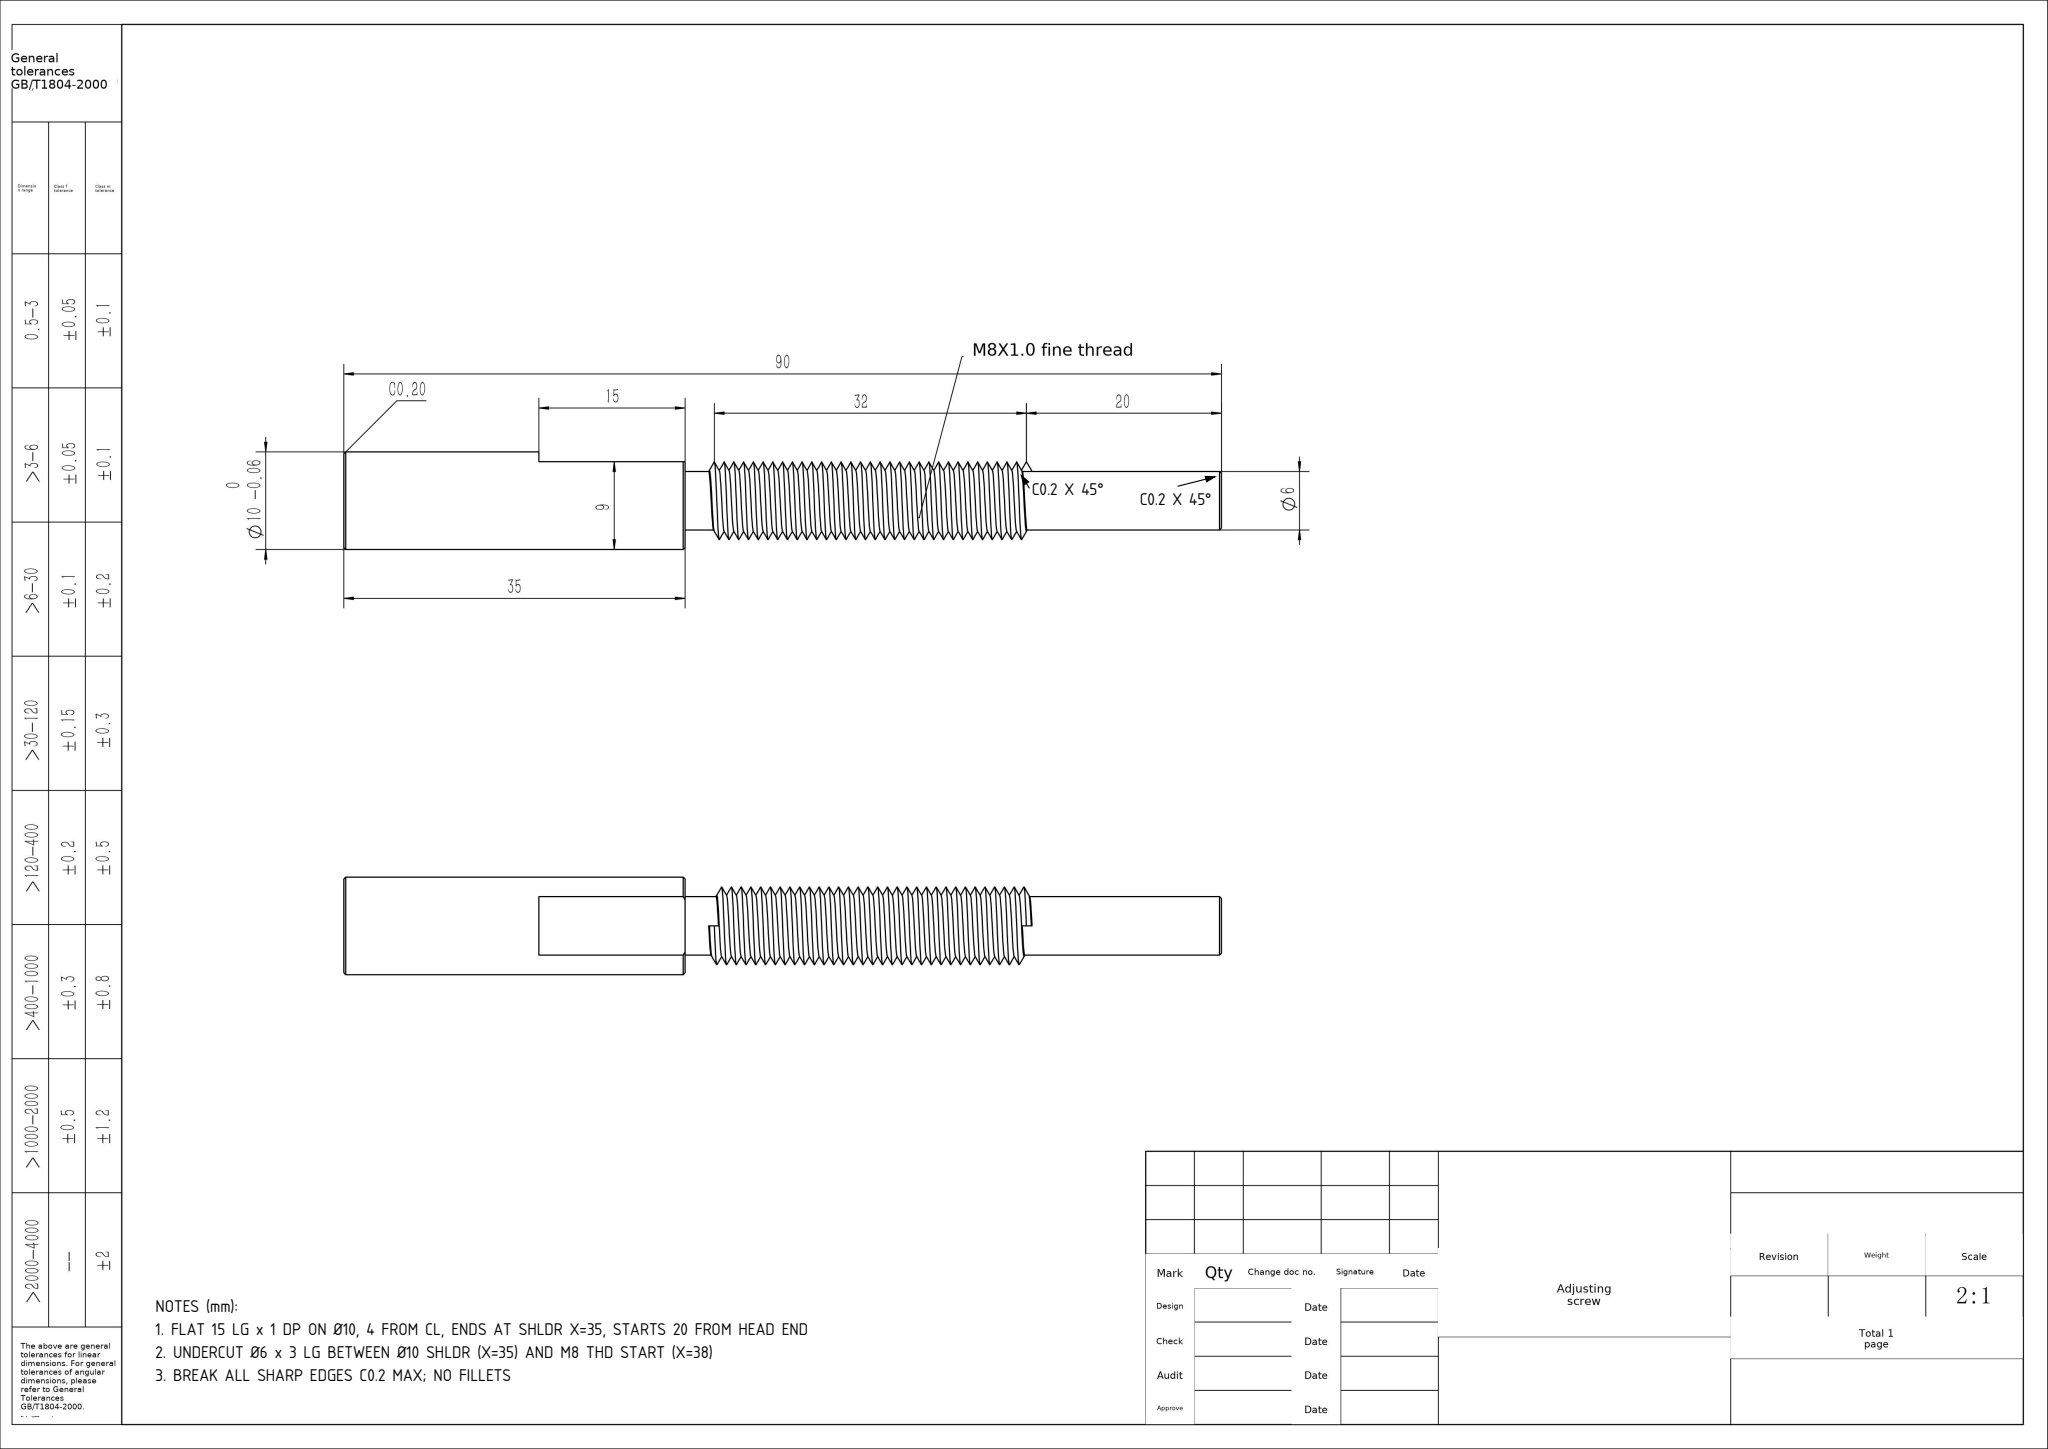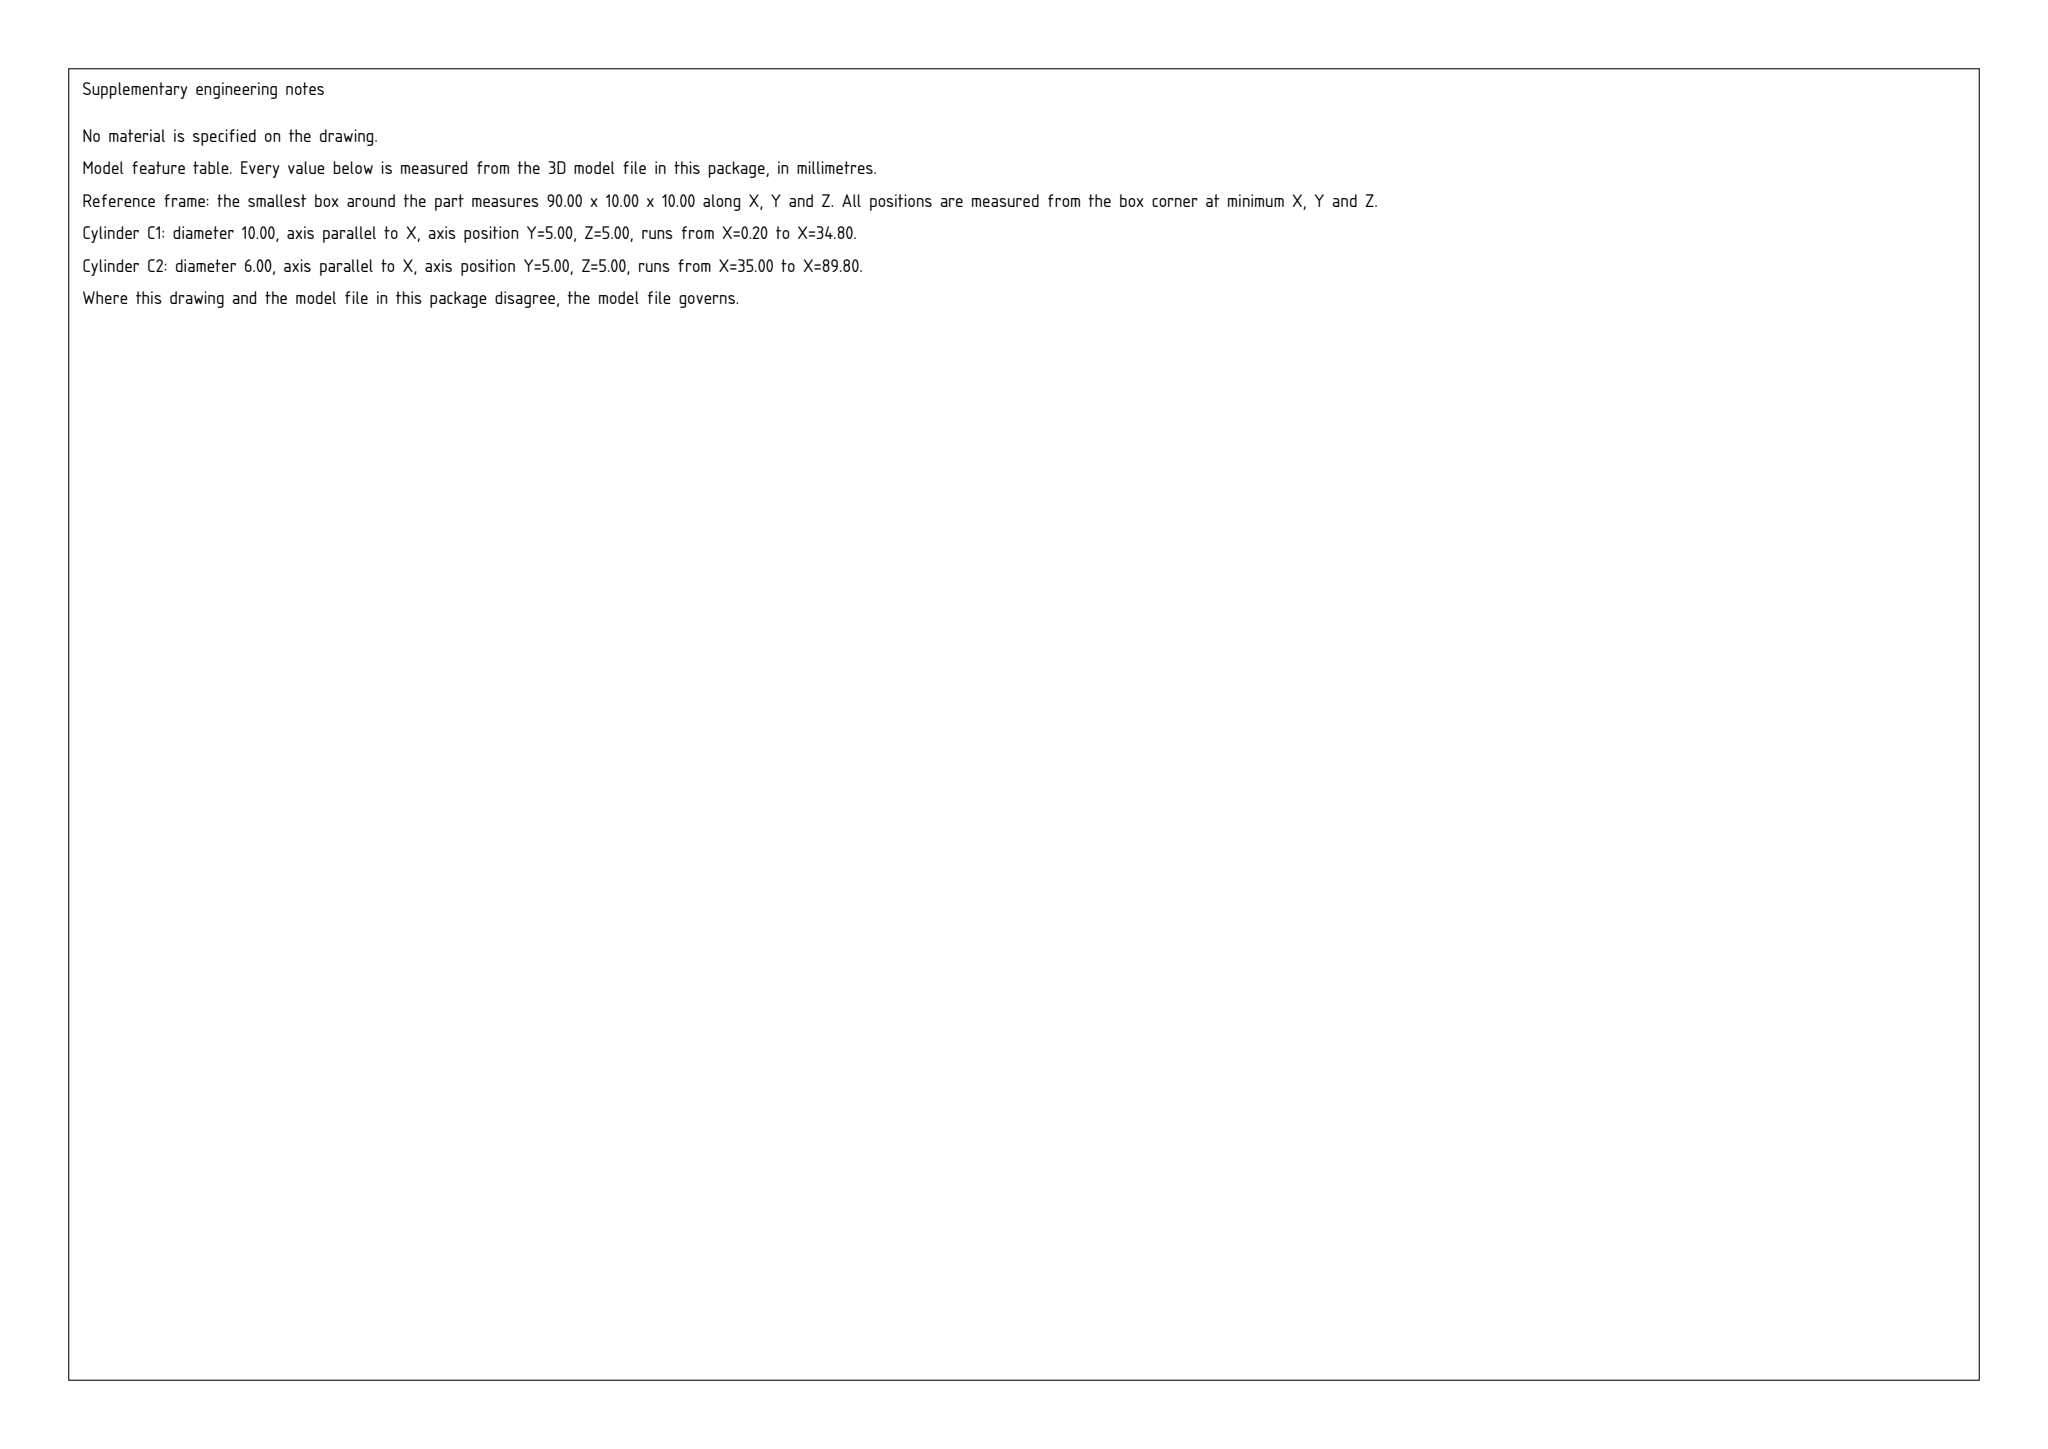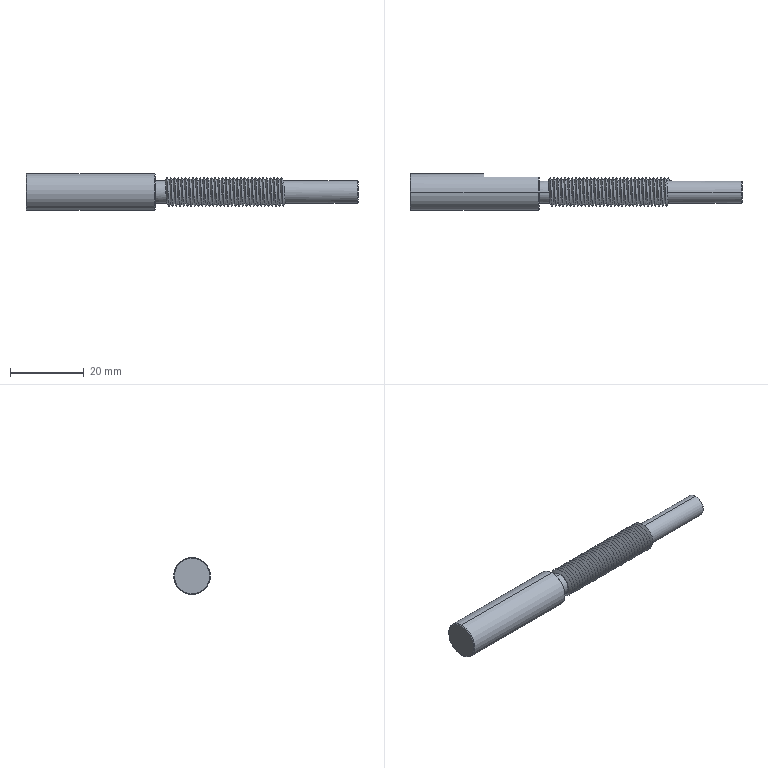Part | SolidWorks | mm | material Plain Carbon Steel | 1 solid | 24 faces | box 90 x 10 x 10 mm | volume 4625 mm3 | cone 7 | plane 7 | cylinder 6 | spline 4 | commonest cylinder face diameters 6 x4 10 x2
Drawing notes:
FLAT 15 LG x 1 DP ON Ø10, 4 FROM CL, ENDS AT SHLDR X=35, STARTS 20 FROM HEAD END | from the solid: axis plane y=9.0 vs cyl axis y=5.0 (1 deep, 4 from CL); bound by planes x=20 and x=35
UNDERCUT Ø6 x 3 LG BETWEEN Ø10 SHLDR (X=35) AND M8 THD START (X=38) | from the solid: Ø6 x-axis cyl L=3.17 between plane x=35 and thread start x=38; 90-35-32-20=3
C0.2 X 45° AT THD RUNOUT TO Ø6 | from the solid: cone 90° incl, ref dia 5.6 on Ø6 (6->5.6 = 0.2 x 45°)
C0.2 X 45° ON Ø6 FREE END (X=90) | from the solid: 2nd cone 90° incl, ref dia 5.6 at x=90 end plane
BREAK ALL SHARP EDGES C0.2 MAX; NO FILLETS | from the solid: no fillet radii in model; all cones 90° incl giving 0.2 chamfers (Ø10->9.6, Ø6->5.6)